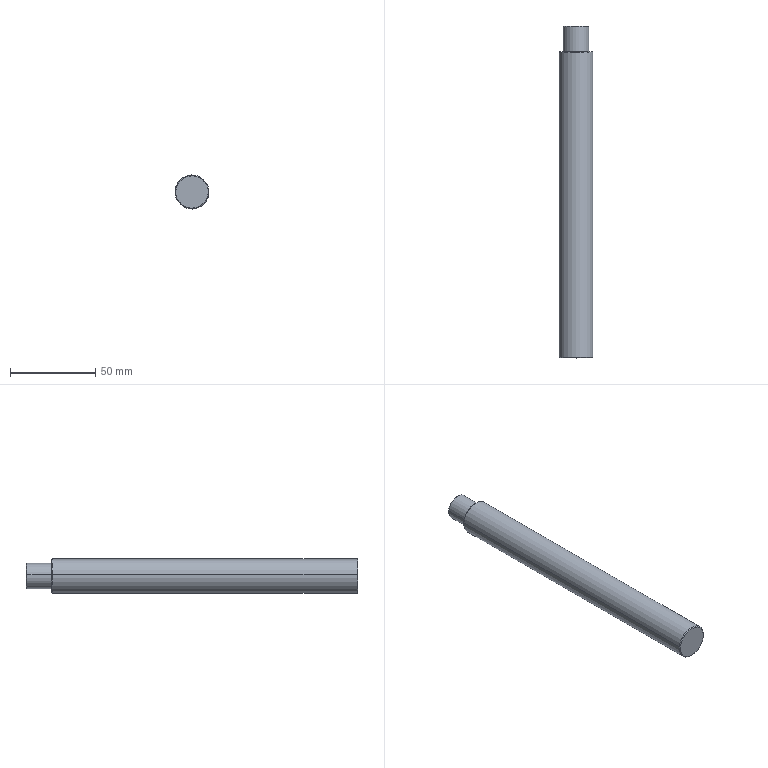Component | SolidWorks | E005GuideAxis-2 | 1 solid | 17 faces | box 20 x 195 x 20 mm | volume 58436 mm3 | cone 8 | cylinder 6 | plane 3 | commonest cylinder face diameters 6.8 x2 15 x2 20 x2 | material Stainless Steel (Ferritic)
build123d program:
from build123d import *

# Parameters (mm, degrees)
SKETCH1_R             = 10
BOSS_EXTRUDE1_DEPTH   = 195
SKETCH2_OUTSIDE_W     = 61.408
SKETCH2_OUTSIDE_H     = 61.408
SKETCH2_OUTSIDE_R     = 7.5
CUT_EXTRUDE1_DEPTH    = 15
M8_TAPPED_HOLE1_D     = 6.8
M8_TAPPED_HOLE1_DEPTH = 19.75
M8_TAPPED_HOLE1_TIP   = 2.043
CHAMFER1_SIZE         = 0.5


with BuildPart() as part:
    # Sketch1 → Boss-Extrude1 (new body)
    with BuildSketch(Plane.XY):
        Circle(SKETCH1_R)
    extrude(amount=BOSS_EXTRUDE1_DEPTH)

    # Sketch2 outside → Cut-Extrude1 (cut)
    with BuildSketch(Plane.XY.offset(195)):
        Rectangle(SKETCH2_OUTSIDE_W, SKETCH2_OUTSIDE_H)
        Circle(SKETCH2_OUTSIDE_R, mode=Mode.SUBTRACT)
    extrude(amount=-CUT_EXTRUDE1_DEPTH, mode=Mode.SUBTRACT)

    # M8 Tapped Hole1
    with Locations(Plane.XY.offset(195)):
        with Locations((0, 0)):
            Hole(M8_TAPPED_HOLE1_D / 2, depth=M8_TAPPED_HOLE1_DEPTH)
            with Locations((0, 0, -(M8_TAPPED_HOLE1_DEPTH + M8_TAPPED_HOLE1_TIP / 2))):  # 118° drill point
                Cone(0, M8_TAPPED_HOLE1_D / 2, M8_TAPPED_HOLE1_TIP, mode=Mode.SUBTRACT)

    # Chamfer1
    chamfer1_edges = [part.edges().sort_by_distance(p)[0] for p in [
        (-7.5, 0, 195),
        (-10, 0, 0),
        (-10, 0, 180),
    ]]
    chamfer(chamfer1_edges, length=CHAMFER1_SIZE)


solid = part.part

# Placed as in the assembly
solid = solid.moved(Location((91, 101, 0), (-90, 0, 0)))
STEP:
#1=COLOUR_RGB('',0.7922,0.8196,0.9333);
#2=FILL_AREA_STYLE_COLOUR('',#1);
#3=FILL_AREA_STYLE('',(#2));
#4=SURFACE_STYLE_FILL_AREA(#3);
#5=SURFACE_SIDE_STYLE('',(#4));
#6=SURFACE_STYLE_USAGE(.BOTH.,#5);
#7=PRESENTATION_STYLE_ASSIGNMENT((#6));
#8=CARTESIAN_POINT('',(3.857,11.654,-0.02823));
#9=VERTEX_POINT('',#8);
#10=CARTESIAN_POINT('',(3.309,11.654,0.02823));
#11=VERTEX_POINT('',#10);
#12=CARTESIAN_POINT('',(3.583,11.654,-0.));
#13=DIRECTION('',(0.,1.,0.));
#14=DIRECTION('',(0.9947,0.,-0.1024));
#15=AXIS2_PLACEMENT_3D('',#12,#13,#14);
#16=CIRCLE('',#15,0.2756);
#17=EDGE_CURVE('',#9,#11,#16,.T.);
#18=ORIENTED_EDGE('',*,*,#17,.F.);
#19=CARTESIAN_POINT('',(3.876,11.634,-0.03024));
#20=VERTEX_POINT('',#19);
#21=CARTESIAN_POINT('',(3.857,11.654,-0.02823));
#22=DIRECTION('',(0.7034,-0.7071,-0.07242));
#23=VECTOR('',#22,39.37);
#24=LINE('',#21,#23);
#25=EDGE_CURVE('',#9,#20,#24,.T.);
#26=ORIENTED_EDGE('',*,*,#25,.T.);
#27=CARTESIAN_POINT('',(3.289,11.634,0.03024));
#28=VERTEX_POINT('',#27);
#29=CARTESIAN_POINT('',(3.583,11.634,-0.));
#30=DIRECTION('',(0.,-1.,0.));
#31=DIRECTION('',(0.9947,0.,-0.1024));
#32=AXIS2_PLACEMENT_3D('',#29,#30,#31);
#33=CIRCLE('',#32,0.2953);
#34=EDGE_CURVE('',#28,#20,#33,.T.);
#35=ORIENTED_EDGE('',*,*,#34,.F.);
#36=CARTESIAN_POINT('',(3.309,11.654,0.02823));
#37=DIRECTION('',(-0.7034,-0.7071,0.07242));
#38=VECTOR('',#37,39.37);
#39=LINE('',#36,#38);
#40=EDGE_CURVE('',#11,#28,#39,.T.);
#41=ORIENTED_EDGE('',*,*,#40,.F.);
#42=EDGE_LOOP('',(#18,#26,#35,#41));
#43=FACE_OUTER_BOUND('',#42,.T.);
#44=CARTESIAN_POINT('',(3.583,11.654,-0.));
#45=DIRECTION('',(0.,-1.,0.));
#46=DIRECTION('',(-0.9947,0.,0.1024));
#47=AXIS2_PLACEMENT_3D('',#44,#45,#46);
#48=CONICAL_SURFACE('',#47,0.2756,0.7854);
#49=ADVANCED_FACE('',(#43),#48,.T.);
#50=CARTESIAN_POINT('',(3.955,11.063,-0.03831));
#51=VERTEX_POINT('',#50);
#52=CARTESIAN_POINT('',(3.211,11.063,0.03831));
#53=VERTEX_POINT('',#52);
#54=CARTESIAN_POINT('',(3.583,11.063,-0.));
#55=DIRECTION('',(0.,1.,0.));
#56=DIRECTION('',(0.9947,0.,-0.1024));
#57=AXIS2_PLACEMENT_3D('',#54,#55,#56);
#58=CIRCLE('',#57,0.374);
#59=EDGE_CURVE('',#51,#53,#58,.T.);
#60=ORIENTED_EDGE('',*,*,#59,.F.);
#61=CARTESIAN_POINT('',(3.974,11.043,-0.04032));
#62=VERTEX_POINT('',#61);
#63=CARTESIAN_POINT('',(3.955,11.063,-0.03831));
#64=DIRECTION('',(0.7034,-0.7071,-0.07242));
#65=VECTOR('',#64,39.37);
#66=LINE('',#63,#65);
#67=EDGE_CURVE('',#51,#62,#66,.T.);
#68=ORIENTED_EDGE('',*,*,#67,.T.);
#69=CARTESIAN_POINT('',(3.191,11.043,0.04032));
#70=VERTEX_POINT('',#69);
#71=CARTESIAN_POINT('',(3.583,11.043,-0.));
#72=DIRECTION('',(0.,-1.,0.));
#73=DIRECTION('',(0.9947,0.,-0.1024));
#74=AXIS2_PLACEMENT_3D('',#71,#72,#73);
#75=CIRCLE('',#74,0.3937);
#76=EDGE_CURVE('',#70,#62,#75,.T.);
#77=ORIENTED_EDGE('',*,*,#76,.F.);
#78=CARTESIAN_POINT('',(3.211,11.063,0.03831));
#79=DIRECTION('',(-0.7034,-0.7071,0.07242));
#80=VECTOR('',#79,39.37);
#81=LINE('',#78,#80);
#82=EDGE_CURVE('',#53,#70,#81,.T.);
#83=ORIENTED_EDGE('',*,*,#82,.F.);
#84=EDGE_LOOP('',(#60,#68,#77,#83));
#85=FACE_OUTER_BOUND('',#84,.T.);
#86=CARTESIAN_POINT('',(3.583,11.063,-0.));
#87=DIRECTION('',(0.,-1.,0.));
#88=DIRECTION('',(-0.9947,0.,0.1024));
#89=AXIS2_PLACEMENT_3D('',#86,#87,#88);
#90=CONICAL_SURFACE('',#89,0.374,0.7854);
#91=ADVANCED_FACE('',(#85),#90,.T.);
#92=CARTESIAN_POINT('',(3.211,3.976,0.03831));
#93=VERTEX_POINT('',#92);
#94=CARTESIAN_POINT('',(3.955,3.976,-0.03831));
#95=VERTEX_POINT('',#94);
#96=CARTESIAN_POINT('',(3.583,3.976,-0.));
#97=DIRECTION('',(0.,-1.,0.));
#98=DIRECTION('',(0.9947,0.,-0.1024));
#99=AXIS2_PLACEMENT_3D('',#96,#97,#98);
#100=CIRCLE('',#99,0.374);
#101=EDGE_CURVE('',#93,#95,#100,.T.);
#102=ORIENTED_EDGE('',*,*,#101,.F.);
#103=CARTESIAN_POINT('',(3.191,3.996,0.04032));
#104=VERTEX_POINT('',#103);
#105=CARTESIAN_POINT('',(3.191,3.996,0.04032));
#106=DIRECTION('',(-0.7034,0.7071,0.07242));
#107=VECTOR('',#106,39.37);
#108=LINE('',#105,#107);
#109=EDGE_CURVE('',#93,#104,#108,.T.);
#110=ORIENTED_EDGE('',*,*,#109,.T.);
#111=CARTESIAN_POINT('',(3.974,3.996,-0.04032));
#112=VERTEX_POINT('',#111);
#113=CARTESIAN_POINT('',(3.583,3.996,-0.));
#114=DIRECTION('',(0.,1.,0.));
#115=DIRECTION('',(0.9947,0.,-0.1024));
#116=AXIS2_PLACEMENT_3D('',#113,#114,#115);
#117=CIRCLE('',#116,0.3937);
#118=EDGE_CURVE('',#112,#104,#117,.T.);
#119=ORIENTED_EDGE('',*,*,#118,.F.);
#120=CARTESIAN_POINT('',(3.974,3.996,-0.04032));
#121=DIRECTION('',(0.7034,0.7071,-0.07242));
#122=VECTOR('',#121,39.37);
#123=LINE('',#120,#122);
#124=EDGE_CURVE('',#95,#112,#123,.T.);
#125=ORIENTED_EDGE('',*,*,#124,.F.);
#126=EDGE_LOOP('',(#102,#110,#119,#125));
#127=FACE_OUTER_BOUND('',#126,.T.);
#128=CARTESIAN_POINT('',(3.583,3.996,-0.));
#129=DIRECTION('',(0.,1.,0.));
#130=DIRECTION('',(0.9947,0.,-0.1024));
#131=AXIS2_PLACEMENT_3D('',#128,#129,#130);
#132=CONICAL_SURFACE('',#131,0.3937,0.7854);
#133=ADVANCED_FACE('',(#127),#132,.T.);
#134=CARTESIAN_POINT('',(3.45,10.876,0.01371));
#135=VERTEX_POINT('',#134);
#136=CARTESIAN_POINT('',(3.716,10.876,-0.01371));
#137=VERTEX_POINT('',#136);
#138=CARTESIAN_POINT('',(3.583,10.876,-0.));
#139=DIRECTION('',(0.,1.,0.));
#140=DIRECTION('',(0.9947,0.,-0.1024));
#141=AXIS2_PLACEMENT_3D('',#138,#139,#140);
#142=CIRCLE('',#141,0.1339);
#143=EDGE_CURVE('',#135,#137,#142,.T.);
#144=ORIENTED_EDGE('',*,*,#143,.F.);
#145=CARTESIAN_POINT('',(3.45,11.654,0.01371));
#146=VERTEX_POINT('',#145);
#147=CARTESIAN_POINT('',(3.45,11.654,0.01371));
#148=DIRECTION('',(0.,1.,0.));
#149=VECTOR('',#148,39.37);
#150=LINE('',#147,#149);
#151=EDGE_CURVE('',#135,#146,#150,.T.);
#152=ORIENTED_EDGE('',*,*,#151,.T.);
#153=CARTESIAN_POINT('',(3.716,11.654,-0.01371));
#154=VERTEX_POINT('',#153);
#155=CARTESIAN_POINT('',(3.583,11.654,-0.));
#156=DIRECTION('',(0.,1.,0.));
#157=DIRECTION('',(0.9947,0.,-0.1024));
#158=AXIS2_PLACEMENT_3D('',#155,#156,#157);
#159=CIRCLE('',#158,0.1339);
#160=EDGE_CURVE('',#146,#154,#159,.T.);
#161=ORIENTED_EDGE('',*,*,#160,.T.);
#162=CARTESIAN_POINT('',(3.716,11.654,-0.01371));
#163=DIRECTION('',(0.,1.,0.));
#164=VECTOR('',#163,39.37);
#165=LINE('',#162,#164);
#166=EDGE_CURVE('',#137,#154,#165,.T.);
#167=ORIENTED_EDGE('',*,*,#166,.F.);
#168=EDGE_LOOP('',(#144,#152,#161,#167));
#169=FACE_OUTER_BOUND('',#168,.T.);
#170=CARTESIAN_POINT('',(3.583,11.654,-0.));
#171=DIRECTION('',(0.,1.,0.));
#172=DIRECTION('',(0.9947,0.,-0.1024));
#173=AXIS2_PLACEMENT_3D('',#170,#171,#172);
#174=CYLINDRICAL_SURFACE('',#173,0.1339);
#175=ADVANCED_FACE('',(#169),#174,.F.);
#176=CARTESIAN_POINT('',(3.583,10.796,-0.));
#177=VERTEX_POINT('',#176);
#178=CARTESIAN_POINT('',(3.716,10.876,-0.01371));
#179=DIRECTION('',(0.8527,0.515,-0.08779));
#180=VECTOR('',#179,39.37);
#181=LINE('',#178,#180);
#182=EDGE_CURVE('',#177,#137,#181,.T.);
#183=ORIENTED_EDGE('',*,*,#182,.F.);
#184=CARTESIAN_POINT('',(3.45,10.876,0.01371));
#185=DIRECTION('',(-0.8527,0.515,0.08779));
#186=VECTOR('',#185,39.37);
#187=LINE('',#184,#186);
#188=EDGE_CURVE('',#177,#135,#187,.T.);
#189=ORIENTED_EDGE('',*,*,#188,.T.);
#190=ORIENTED_EDGE('',*,*,#143,.T.);
#191=EDGE_LOOP('',(#183,#189,#190));
#192=FACE_OUTER_BOUND('',#191,.T.);
#193=CARTESIAN_POINT('',(3.583,10.876,-0.));
#194=DIRECTION('',(0.,1.,0.));
#195=DIRECTION('',(0.9947,0.,-0.1024));
#196=AXIS2_PLACEMENT_3D('',#193,#194,#195);
#197=CONICAL_SURFACE('',#196,0.1339,1.03);
#198=ADVANCED_FACE('',(#192),#197,.F.);
#199=CARTESIAN_POINT('',(3.876,11.063,-0.03024));
#200=VERTEX_POINT('',#199);
#201=CARTESIAN_POINT('',(3.289,11.063,0.03024));
#202=VERTEX_POINT('',#201);
#203=CARTESIAN_POINT('',(3.583,11.063,-0.));
#204=DIRECTION('',(0.,1.,0.));
#205=DIRECTION('',(0.9947,0.,-0.1024));
#206=AXIS2_PLACEMENT_3D('',#203,#204,#205);
#207=CIRCLE('',#206,0.2953);
#208=EDGE_CURVE('',#200,#202,#207,.T.);
#209=ORIENTED_EDGE('',*,*,#208,.T.);
#210=CARTESIAN_POINT('',(3.289,11.063,0.03024));
#211=DIRECTION('',(0.,1.,0.));
#212=VECTOR('',#211,39.37);
#213=LINE('',#210,#212);
#214=EDGE_CURVE('',#202,#28,#213,.T.);
#215=ORIENTED_EDGE('',*,*,#214,.T.);
#216=ORIENTED_EDGE('',*,*,#34,.T.);
#217=CARTESIAN_POINT('',(3.876,11.063,-0.03024));
#218=DIRECTION('',(0.,1.,0.));
#219=VECTOR('',#218,39.37);
#220=LINE('',#217,#219);
#221=EDGE_CURVE('',#200,#20,#220,.T.);
#222=ORIENTED_EDGE('',*,*,#221,.F.);
#223=EDGE_LOOP('',(#209,#215,#216,#222));
#224=FACE_OUTER_BOUND('',#223,.T.);
#225=CARTESIAN_POINT('',(3.583,11.063,-0.));
#226=DIRECTION('',(0.,1.,0.));
#227=DIRECTION('',(0.9947,0.,-0.1024));
#228=AXIS2_PLACEMENT_3D('',#225,#226,#227);
#229=CYLINDRICAL_SURFACE('',#228,0.2953);
#230=ADVANCED_FACE('',(#224),#229,.T.);
#231=ORIENTED_EDGE('',*,*,#76,.T.);
#232=CARTESIAN_POINT('',(3.974,11.654,-0.04032));
#233=DIRECTION('',(0.,-1.,0.));
#234=VECTOR('',#233,39.37);
#235=LINE('',#232,#234);
#236=EDGE_CURVE('',#62,#112,#235,.T.);
#237=ORIENTED_EDGE('',*,*,#236,.T.);
#238=ORIENTED_EDGE('',*,*,#118,.T.);
#239=CARTESIAN_POINT('',(3.191,11.654,0.04032));
#240=DIRECTION('',(0.,-1.,0.));
#241=VECTOR('',#240,39.37);
#242=LINE('',#239,#241);
#243=EDGE_CURVE('',#70,#104,#242,.T.);
#244=ORIENTED_EDGE('',*,*,#243,.F.);
#245=EDGE_LOOP('',(#231,#237,#238,#244));
#246=FACE_OUTER_BOUND('',#245,.T.);
#247=CARTESIAN_POINT('',(3.583,11.654,-0.));
#248=DIRECTION('',(0.,-1.,0.));
#249=DIRECTION('',(-0.9947,0.,0.1024));
#250=AXIS2_PLACEMENT_3D('',#247,#248,#249);
#251=CYLINDRICAL_SURFACE('',#250,0.3937);
#252=ADVANCED_FACE('',(#246),#251,.T.);
#253=ORIENTED_EDGE('',*,*,#236,.F.);
#254=CARTESIAN_POINT('',(3.583,11.043,-0.));
#255=DIRECTION('',(0.,-1.,0.));
#256=DIRECTION('',(0.9947,0.,-0.1024));
#257=AXIS2_PLACEMENT_3D('',#254,#255,#256);
#258=CIRCLE('',#257,0.3937);
#259=EDGE_CURVE('',#62,#70,#258,.T.);
#260=ORIENTED_EDGE('',*,*,#259,.T.);
#261=ORIENTED_EDGE('',*,*,#243,.T.);
#262=CARTESIAN_POINT('',(3.583,3.996,-0.));
#263=DIRECTION('',(0.,1.,0.));
#264=DIRECTION('',(0.9947,0.,-0.1024));
#265=AXIS2_PLACEMENT_3D('',#262,#263,#264);
#266=CIRCLE('',#265,0.3937);
#267=EDGE_CURVE('',#104,#112,#266,.T.);
#268=ORIENTED_EDGE('',*,*,#267,.T.);
#269=EDGE_LOOP('',(#253,#260,#261,#268));
#270=FACE_OUTER_BOUND('',#269,.T.);
#271=CARTESIAN_POINT('',(3.583,11.654,-0.));
#272=DIRECTION('',(0.,-1.,0.));
#273=DIRECTION('',(-0.9947,0.,0.1024));
#274=AXIS2_PLACEMENT_3D('',#271,#272,#273);
#275=CYLINDRICAL_SURFACE('',#274,0.3937);
#276=ADVANCED_FACE('',(#270),#275,.T.);
#277=CARTESIAN_POINT('',(3.583,3.976,-0.));
#278=DIRECTION('',(0.,-1.,0.));
#279=DIRECTION('',(0.9947,0.,-0.1024));
#280=AXIS2_PLACEMENT_3D('',#277,#278,#279);
#281=CIRCLE('',#280,0.374);
#282=EDGE_CURVE('',#95,#93,#281,.T.);
#283=ORIENTED_EDGE('',*,*,#282,.T.);
#284=ORIENTED_EDGE('',*,*,#101,.T.);
#285=EDGE_LOOP('',(#283,#284));
#286=FACE_OUTER_BOUND('',#285,.T.);
#287=CARTESIAN_POINT('',(3.583,3.976,-0.));
#288=DIRECTION('',(0.,1.,0.));
#289=DIRECTION('',(0.9947,0.,-0.1024));
#290=AXIS2_PLACEMENT_3D('',#287,#288,#289);
#291=PLANE('',#290);
#292=ADVANCED_FACE('',(#286),#291,.F.);
#293=CARTESIAN_POINT('',(3.583,11.063,-0.));
#294=DIRECTION('',(0.,1.,0.));
#295=DIRECTION('',(0.9947,0.,-0.1024));
#296=AXIS2_PLACEMENT_3D('',#293,#294,#295);
#297=CIRCLE('',#296,0.374);
#298=EDGE_CURVE('',#53,#51,#297,.T.);
#299=ORIENTED_EDGE('',*,*,#298,.T.);
#300=ORIENTED_EDGE('',*,*,#59,.T.);
#301=EDGE_LOOP('',(#299,#300));
#302=FACE_OUTER_BOUND('',#301,.T.);
#303=ORIENTED_EDGE('',*,*,#208,.F.);
#304=CARTESIAN_POINT('',(3.583,11.063,-0.));
#305=DIRECTION('',(0.,1.,0.));
#306=DIRECTION('',(0.9947,0.,-0.1024));
#307=AXIS2_PLACEMENT_3D('',#304,#305,#306);
#308=CIRCLE('',#307,0.2953);
#309=EDGE_CURVE('',#202,#200,#308,.T.);
#310=ORIENTED_EDGE('',*,*,#309,.F.);
#311=EDGE_LOOP('',(#303,#310));
#312=FACE_BOUND('',#311,.T.);
#313=CARTESIAN_POINT('',(3.583,11.063,-0.));
#314=DIRECTION('',(0.,1.,0.));
#315=DIRECTION('',(0.9947,0.,-0.1024));
#316=AXIS2_PLACEMENT_3D('',#313,#314,#315);
#317=PLANE('',#316);
#318=ADVANCED_FACE('',(#302,#312),#317,.T.);
#319=ORIENTED_EDGE('',*,*,#214,.F.);
#320=ORIENTED_EDGE('',*,*,#309,.T.);
#321=ORIENTED_EDGE('',*,*,#221,.T.);
#322=CARTESIAN_POINT('',(3.583,11.634,-0.));
#323=DIRECTION('',(0.,-1.,0.));
#324=DIRECTION('',(0.9947,0.,-0.1024));
#325=AXIS2_PLACEMENT_3D('',#322,#323,#324);
#326=CIRCLE('',#325,0.2953);
#327=EDGE_CURVE('',#20,#28,#326,.T.);
#328=ORIENTED_EDGE('',*,*,#327,.T.);
#329=EDGE_LOOP('',(#319,#320,#321,#328));
#330=FACE_OUTER_BOUND('',#329,.T.);
#331=CARTESIAN_POINT('',(3.583,11.063,-0.));
#332=DIRECTION('',(0.,1.,0.));
#333=DIRECTION('',(0.9947,0.,-0.1024));
#334=AXIS2_PLACEMENT_3D('',#331,#332,#333);
#335=CYLINDRICAL_SURFACE('',#334,0.2953);
#336=ADVANCED_FACE('',(#330),#335,.T.);
#337=CARTESIAN_POINT('',(3.583,11.654,-0.));
#338=DIRECTION('',(0.,1.,0.));
#339=DIRECTION('',(0.9947,0.,-0.1024));
#340=AXIS2_PLACEMENT_3D('',#337,#338,#339);
#341=CIRCLE('',#340,0.2756);
#342=EDGE_CURVE('',#11,#9,#341,.T.);
#343=ORIENTED_EDGE('',*,*,#342,.T.);
#344=ORIENTED_EDGE('',*,*,#17,.T.);
#345=EDGE_LOOP('',(#343,#344));
#346=FACE_OUTER_BOUND('',#345,.T.);
#347=CARTESIAN_POINT('',(3.583,11.654,-0.));
#348=DIRECTION('',(0.,1.,0.));
#349=DIRECTION('',(0.9947,0.,-0.1024));
#350=AXIS2_PLACEMENT_3D('',#347,#348,#349);
#351=CIRCLE('',#350,0.1339);
#352=EDGE_CURVE('',#154,#146,#351,.T.);
#353=ORIENTED_EDGE('',*,*,#352,.F.);
#354=ORIENTED_EDGE('',*,*,#160,.F.);
#355=EDGE_LOOP('',(#353,#354));
#356=FACE_BOUND('',#355,.T.);
#357=CARTESIAN_POINT('',(3.583,11.654,-0.));
#358=DIRECTION('',(0.,1.,0.));
#359=DIRECTION('',(0.9947,0.,-0.1024));
#360=AXIS2_PLACEMENT_3D('',#357,#358,#359);
#361=PLANE('',#360);
#362=ADVANCED_FACE('',(#346,#356),#361,.T.);
#363=ORIENTED_EDGE('',*,*,#188,.F.);
#364=ORIENTED_EDGE('',*,*,#182,.T.);
#365=CARTESIAN_POINT('',(3.583,10.876,-0.));
#366=DIRECTION('',(0.,1.,0.));
#367=DIRECTION('',(0.9947,0.,-0.1024));
#368=AXIS2_PLACEMENT_3D('',#365,#366,#367);
#369=CIRCLE('',#368,0.1339);
#370=EDGE_CURVE('',#137,#135,#369,.T.);
#371=ORIENTED_EDGE('',*,*,#370,.T.);
#372=EDGE_LOOP('',(#363,#364,#371));
#373=FACE_OUTER_BOUND('',#372,.T.);
#374=CARTESIAN_POINT('',(3.583,10.876,-0.));
#375=DIRECTION('',(0.,1.,0.));
#376=DIRECTION('',(0.9947,0.,-0.1024));
#377=AXIS2_PLACEMENT_3D('',#374,#375,#376);
#378=CONICAL_SURFACE('',#377,0.1339,1.03);
#379=ADVANCED_FACE('',(#373),#378,.F.);
#380=ORIENTED_EDGE('',*,*,#151,.F.);
#381=ORIENTED_EDGE('',*,*,#370,.F.);
#382=ORIENTED_EDGE('',*,*,#166,.T.);
#383=ORIENTED_EDGE('',*,*,#352,.T.);
#384=EDGE_LOOP('',(#380,#381,#382,#383));
#385=FACE_OUTER_BOUND('',#384,.T.);
#386=CARTESIAN_POINT('',(3.583,11.654,-0.));
#387=DIRECTION('',(0.,1.,0.));
#388=DIRECTION('',(0.9947,0.,-0.1024));
#389=AXIS2_PLACEMENT_3D('',#386,#387,#388);
#390=CYLINDRICAL_SURFACE('',#389,0.1339);
#391=ADVANCED_FACE('',(#385),#390,.F.);
#392=ORIENTED_EDGE('',*,*,#109,.F.);
#393=ORIENTED_EDGE('',*,*,#282,.F.);
#394=ORIENTED_EDGE('',*,*,#124,.T.);
#395=ORIENTED_EDGE('',*,*,#267,.F.);
#396=EDGE_LOOP('',(#392,#393,#394,#395));
#397=FACE_OUTER_BOUND('',#396,.T.);
#398=CARTESIAN_POINT('',(3.583,3.996,-0.));
#399=DIRECTION('',(0.,1.,0.));
#400=DIRECTION('',(0.9947,0.,-0.1024));
#401=AXIS2_PLACEMENT_3D('',#398,#399,#400);
#402=CONICAL_SURFACE('',#401,0.3937,0.7854);
#403=ADVANCED_FACE('',(#397),#402,.T.);
#404=ORIENTED_EDGE('',*,*,#67,.F.);
#405=ORIENTED_EDGE('',*,*,#298,.F.);
#406=ORIENTED_EDGE('',*,*,#82,.T.);
#407=ORIENTED_EDGE('',*,*,#259,.F.);
#408=EDGE_LOOP('',(#404,#405,#406,#407));
#409=FACE_OUTER_BOUND('',#408,.T.);
#410=CARTESIAN_POINT('',(3.583,11.063,-0.));
#411=DIRECTION('',(0.,-1.,0.));
#412=DIRECTION('',(-0.9947,0.,0.1024));
#413=AXIS2_PLACEMENT_3D('',#410,#411,#412);
#414=CONICAL_SURFACE('',#413,0.374,0.7854);
#415=ADVANCED_FACE('',(#409),#414,.T.);
#416=ORIENTED_EDGE('',*,*,#25,.F.);
#417=ORIENTED_EDGE('',*,*,#342,.F.);
#418=ORIENTED_EDGE('',*,*,#40,.T.);
#419=ORIENTED_EDGE('',*,*,#327,.F.);
#420=EDGE_LOOP('',(#416,#417,#418,#419));
#421=FACE_OUTER_BOUND('',#420,.T.);
#422=CARTESIAN_POINT('',(3.583,11.654,-0.));
#423=DIRECTION('',(0.,-1.,0.));
#424=DIRECTION('',(-0.9947,0.,0.1024));
#425=AXIS2_PLACEMENT_3D('',#422,#423,#424);
#426=CONICAL_SURFACE('',#425,0.2756,0.7854);
#427=ADVANCED_FACE('',(#421),#426,.T.);
#428=CLOSED_SHELL('',(#49,#91,#133,#175,#198,#230,#252,#276,#292,#318,#336,#362,#379,#391,#403,#415,#427));
#429=MANIFOLD_SOLID_BREP('',#428);
#430=STYLED_ITEM('',(#7),#429);
#431=PRESENTATION_LAYER_ASSIGNMENT('','',(#430));
#432=(LENGTH_UNIT()NAMED_UNIT(*)SI_UNIT($,.METRE.));
#433=LENGTH_MEASURE_WITH_UNIT(LENGTH_MEASURE(0.0254),#432);
#434=DIMENSIONAL_EXPONENTS(1.,0.,0.,0.,0.,0.,0.);
#435=(CONVERSION_BASED_UNIT('',#433)LENGTH_UNIT()NAMED_UNIT(#434));
#436=UNCERTAINTY_MEASURE_WITH_UNIT(LENGTH_MEASURE(0.00001),#435,'','');
#437=(NAMED_UNIT(*)PLANE_ANGLE_UNIT()SI_UNIT($,.RADIAN.));
#438=(NAMED_UNIT(*)SI_UNIT($,.STERADIAN.)SOLID_ANGLE_UNIT());
#439=(GEOMETRIC_REPRESENTATION_CONTEXT(3)GLOBAL_UNCERTAINTY_ASSIGNED_CONTEXT((#436))GLOBAL_UNIT_ASSIGNED_CONTEXT((#435,#437,#438))REPRESENTATION_CONTEXT('',''));
#440=MECHANICAL_DESIGN_GEOMETRIC_PRESENTATION_REPRESENTATION('',(#430),#439);
#441=CARTESIAN_POINT('',(0.,0.,0.));
#442=DIRECTION('',(0.,0.,1.));
#443=DIRECTION('',(1.,0.,0.));
#444=AXIS2_PLACEMENT_3D('',#441,#442,#443);
#445=(LENGTH_UNIT()NAMED_UNIT(*)SI_UNIT($,.METRE.));
#446=LENGTH_MEASURE_WITH_UNIT(LENGTH_MEASURE(0.0254),#445);
#447=DIMENSIONAL_EXPONENTS(1.,0.,0.,0.,0.,0.,0.);
#448=(CONVERSION_BASED_UNIT('',#446)LENGTH_UNIT()NAMED_UNIT(#447));
#449=UNCERTAINTY_MEASURE_WITH_UNIT(LENGTH_MEASURE(0.00001),#448,'','');
#450=(NAMED_UNIT(*)PLANE_ANGLE_UNIT()SI_UNIT($,.RADIAN.));
#451=(NAMED_UNIT(*)SI_UNIT($,.STERADIAN.)SOLID_ANGLE_UNIT());
#452=(GEOMETRIC_REPRESENTATION_CONTEXT(3)GLOBAL_UNCERTAINTY_ASSIGNED_CONTEXT((#449))GLOBAL_UNIT_ASSIGNED_CONTEXT((#448,#450,#451))REPRESENTATION_CONTEXT('',''));
#453=ADVANCED_BREP_SHAPE_REPRESENTATION('',(#429,#444),#452);